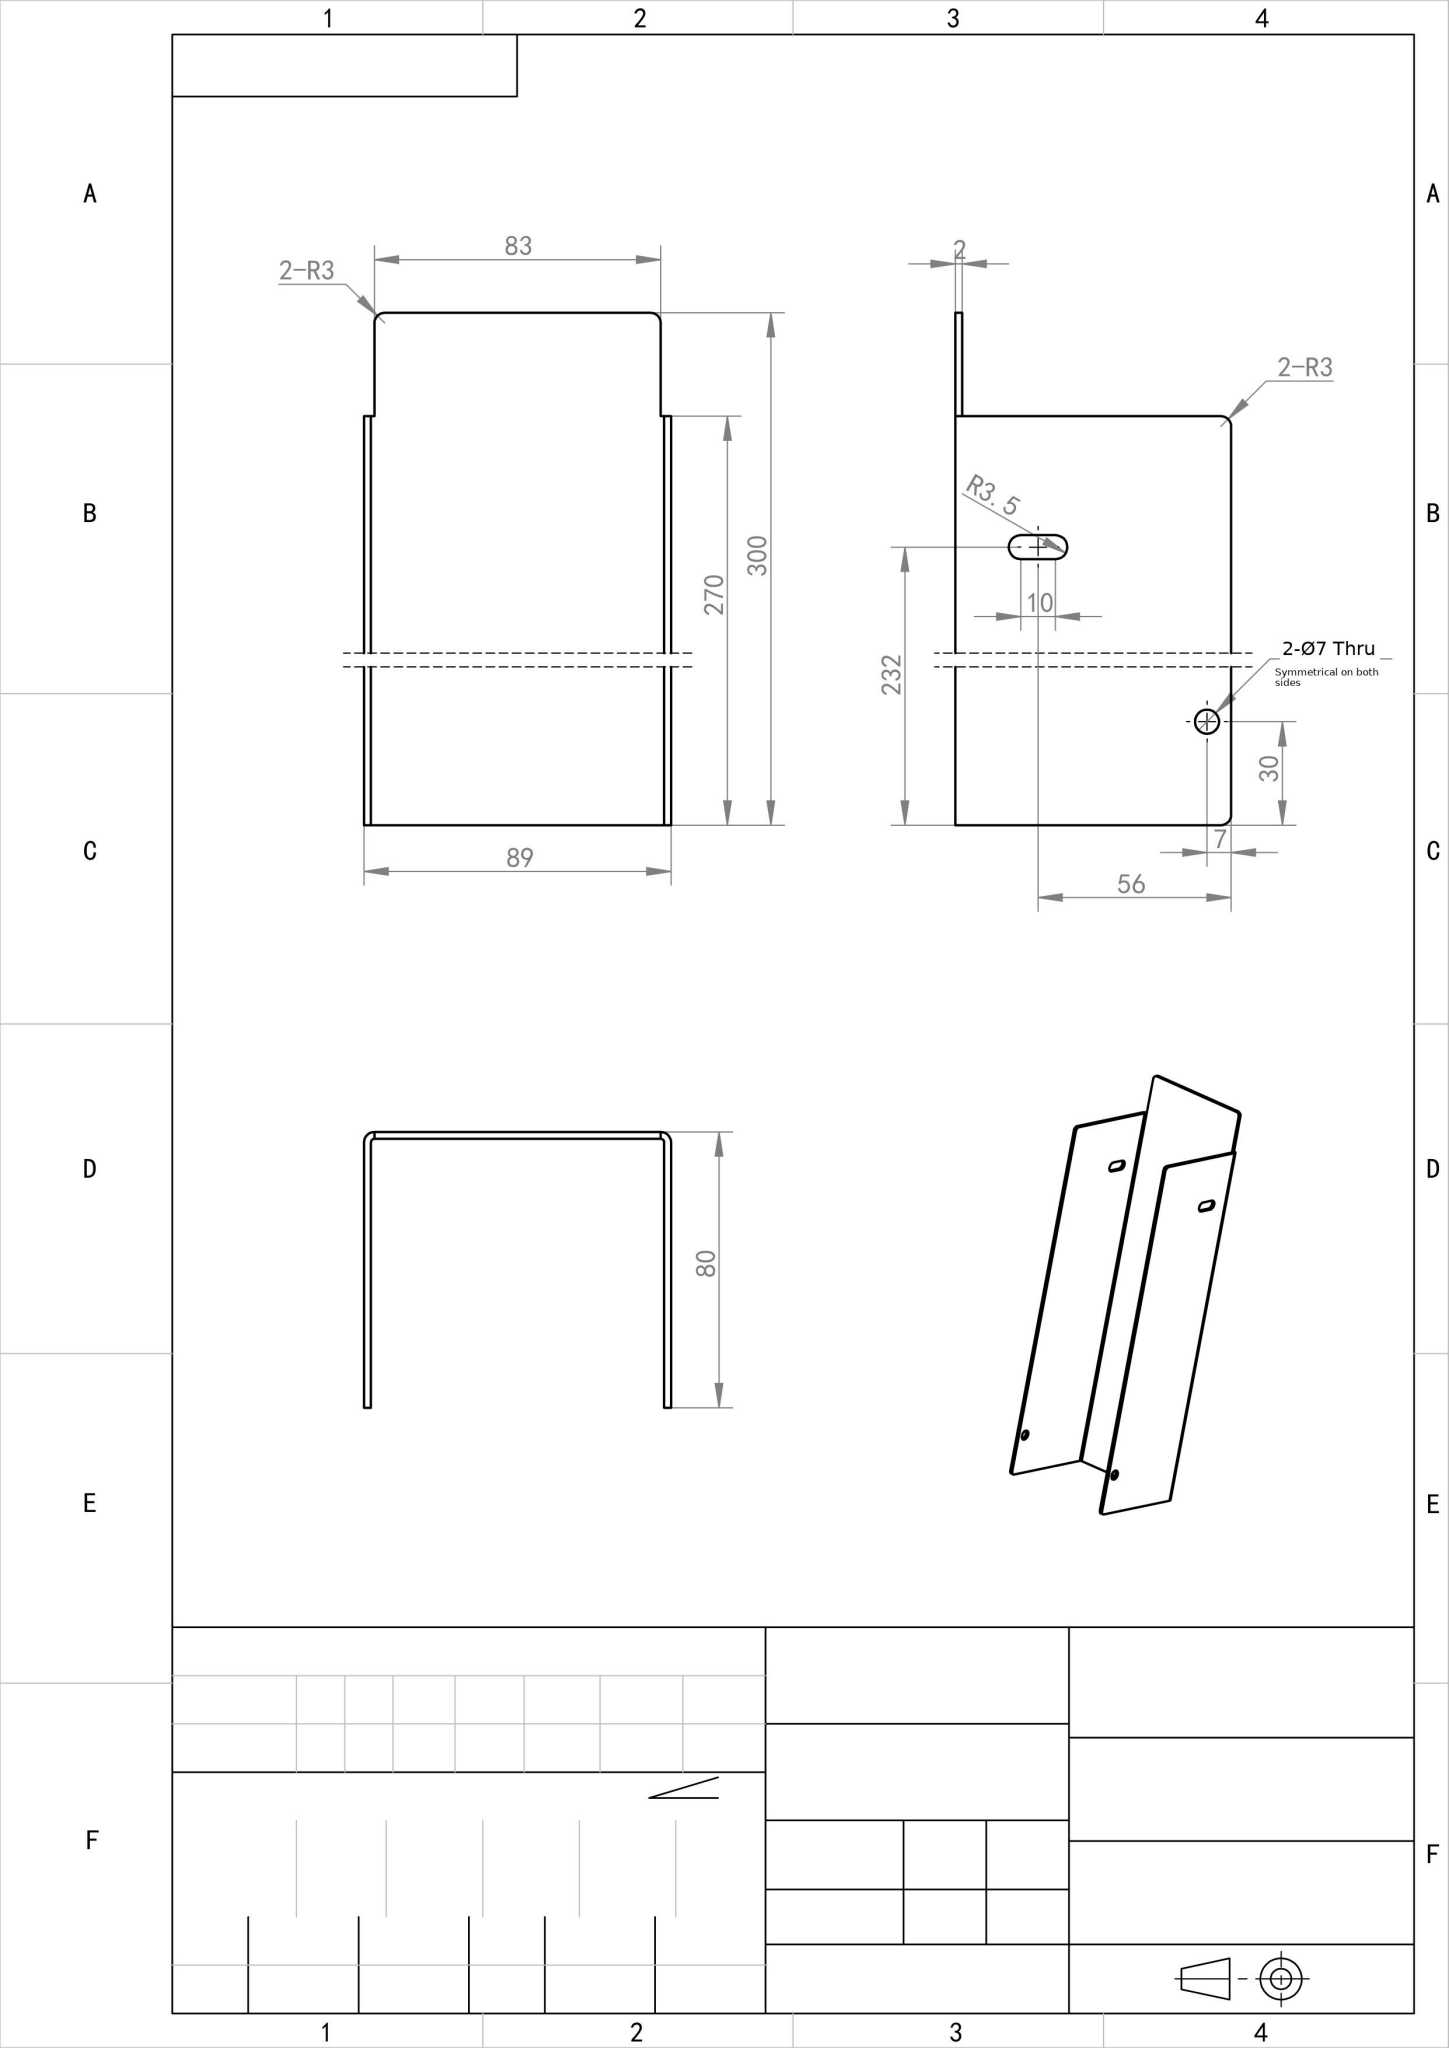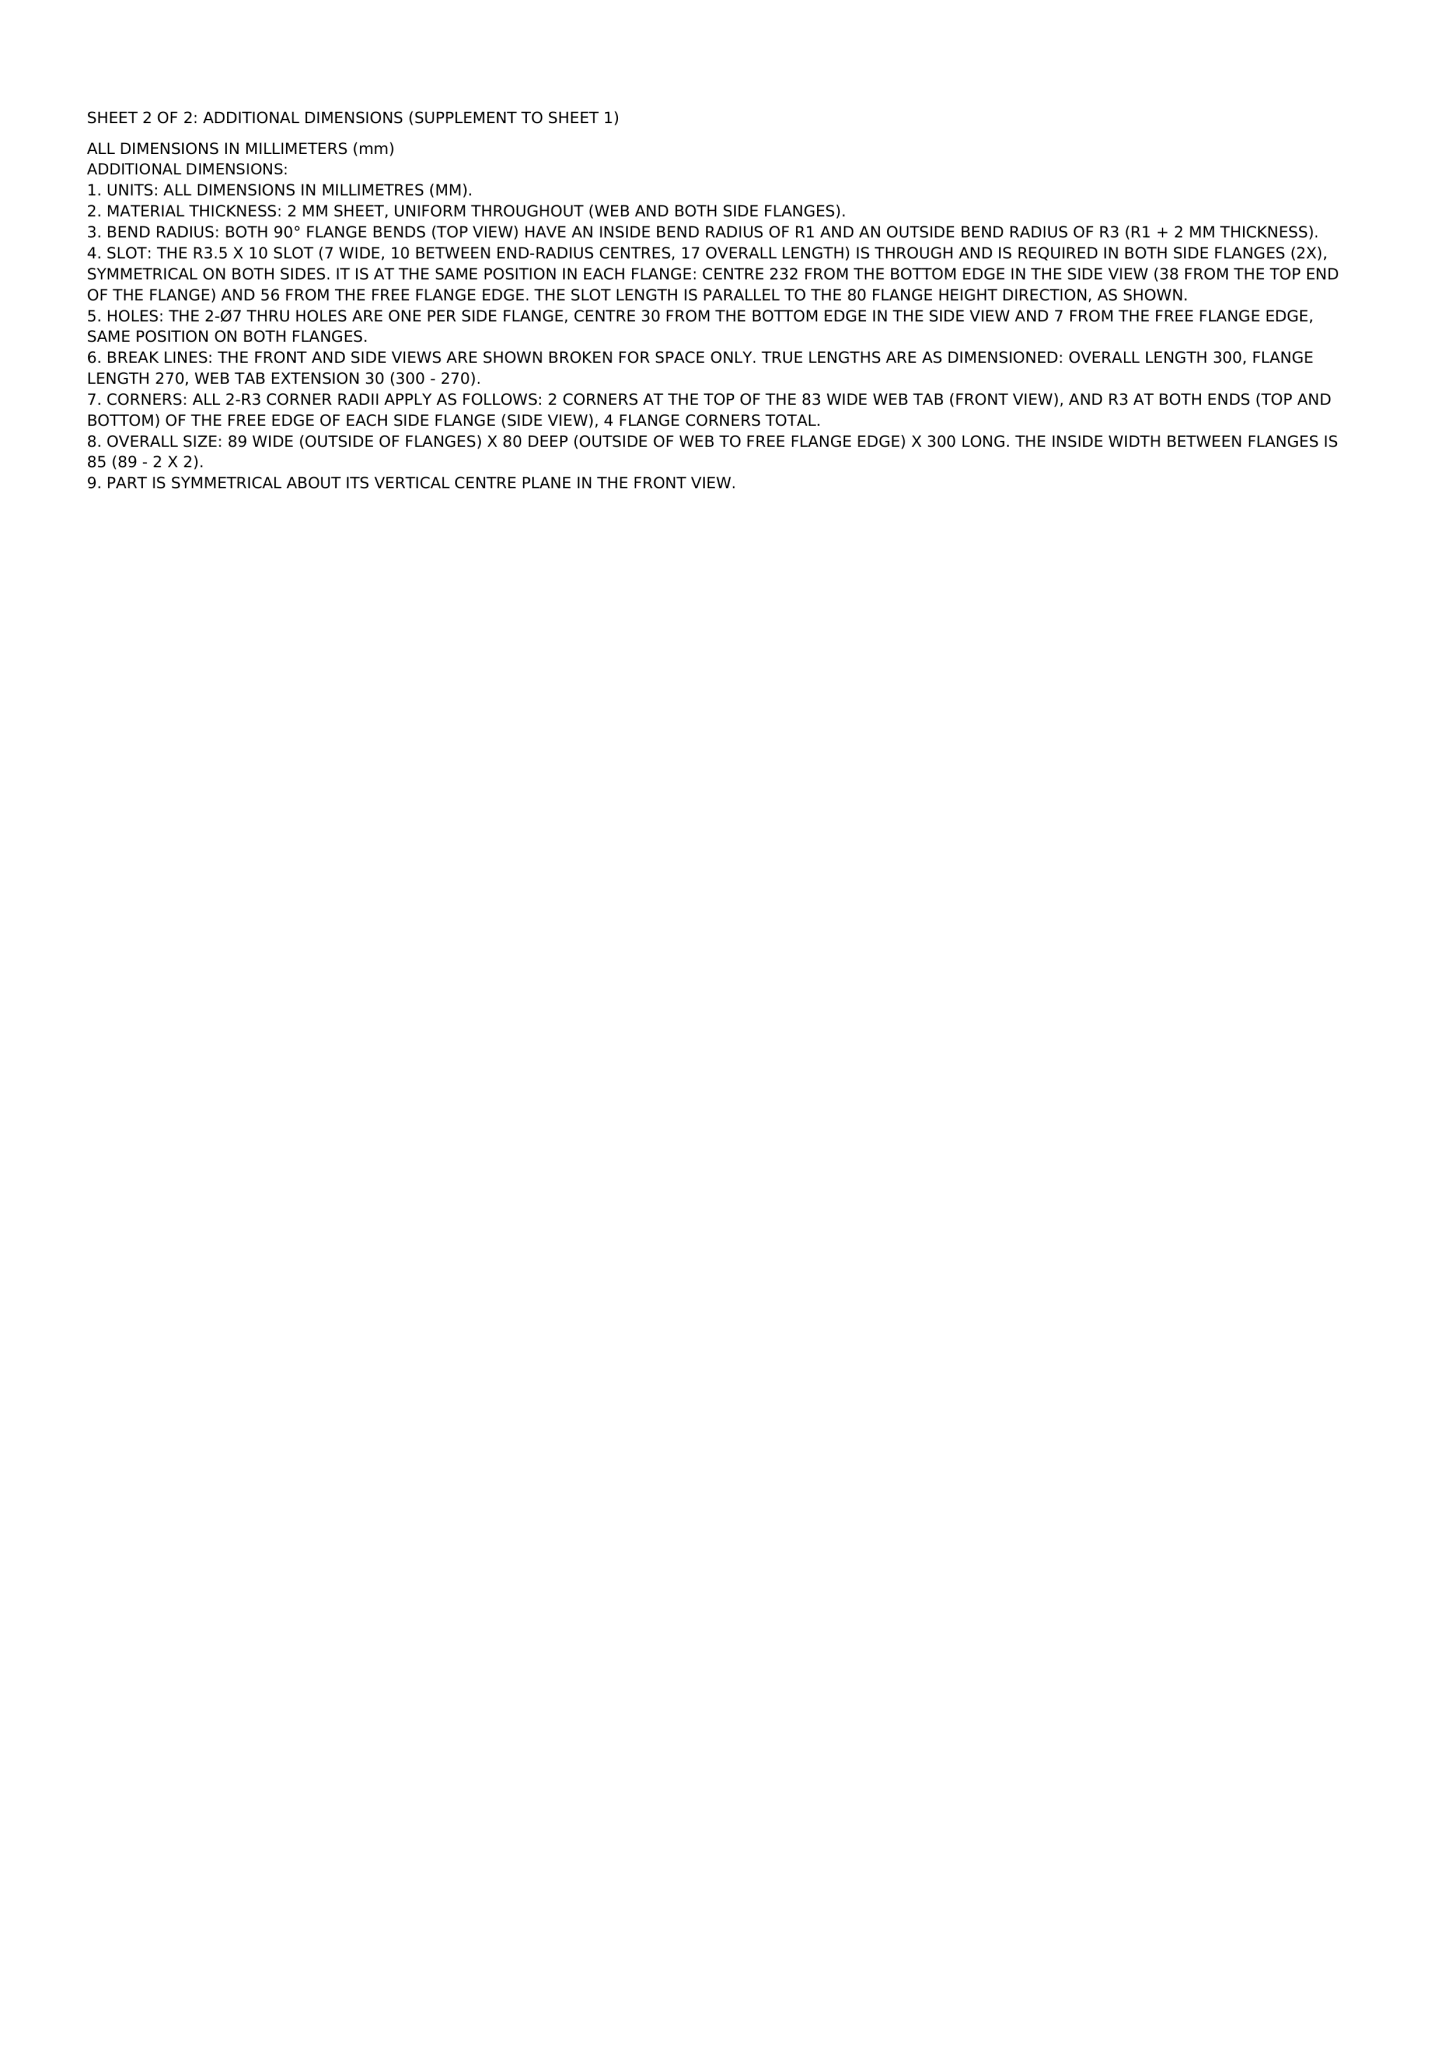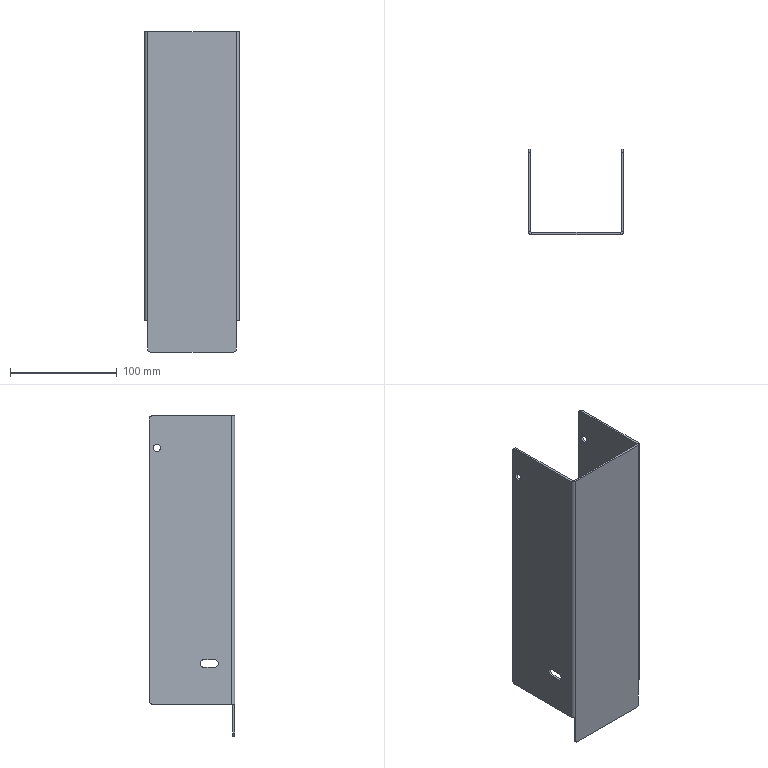Part | NX | mm | U-Shaped Three-Hole Wall Bracket | 1 solid | 44 faces | box 89 x 80 x 300 mm | volume 135742 mm3 | plane 24 | cylinder 20 | commonest cylinder face diameters 7 x10 6 x8 2 x2